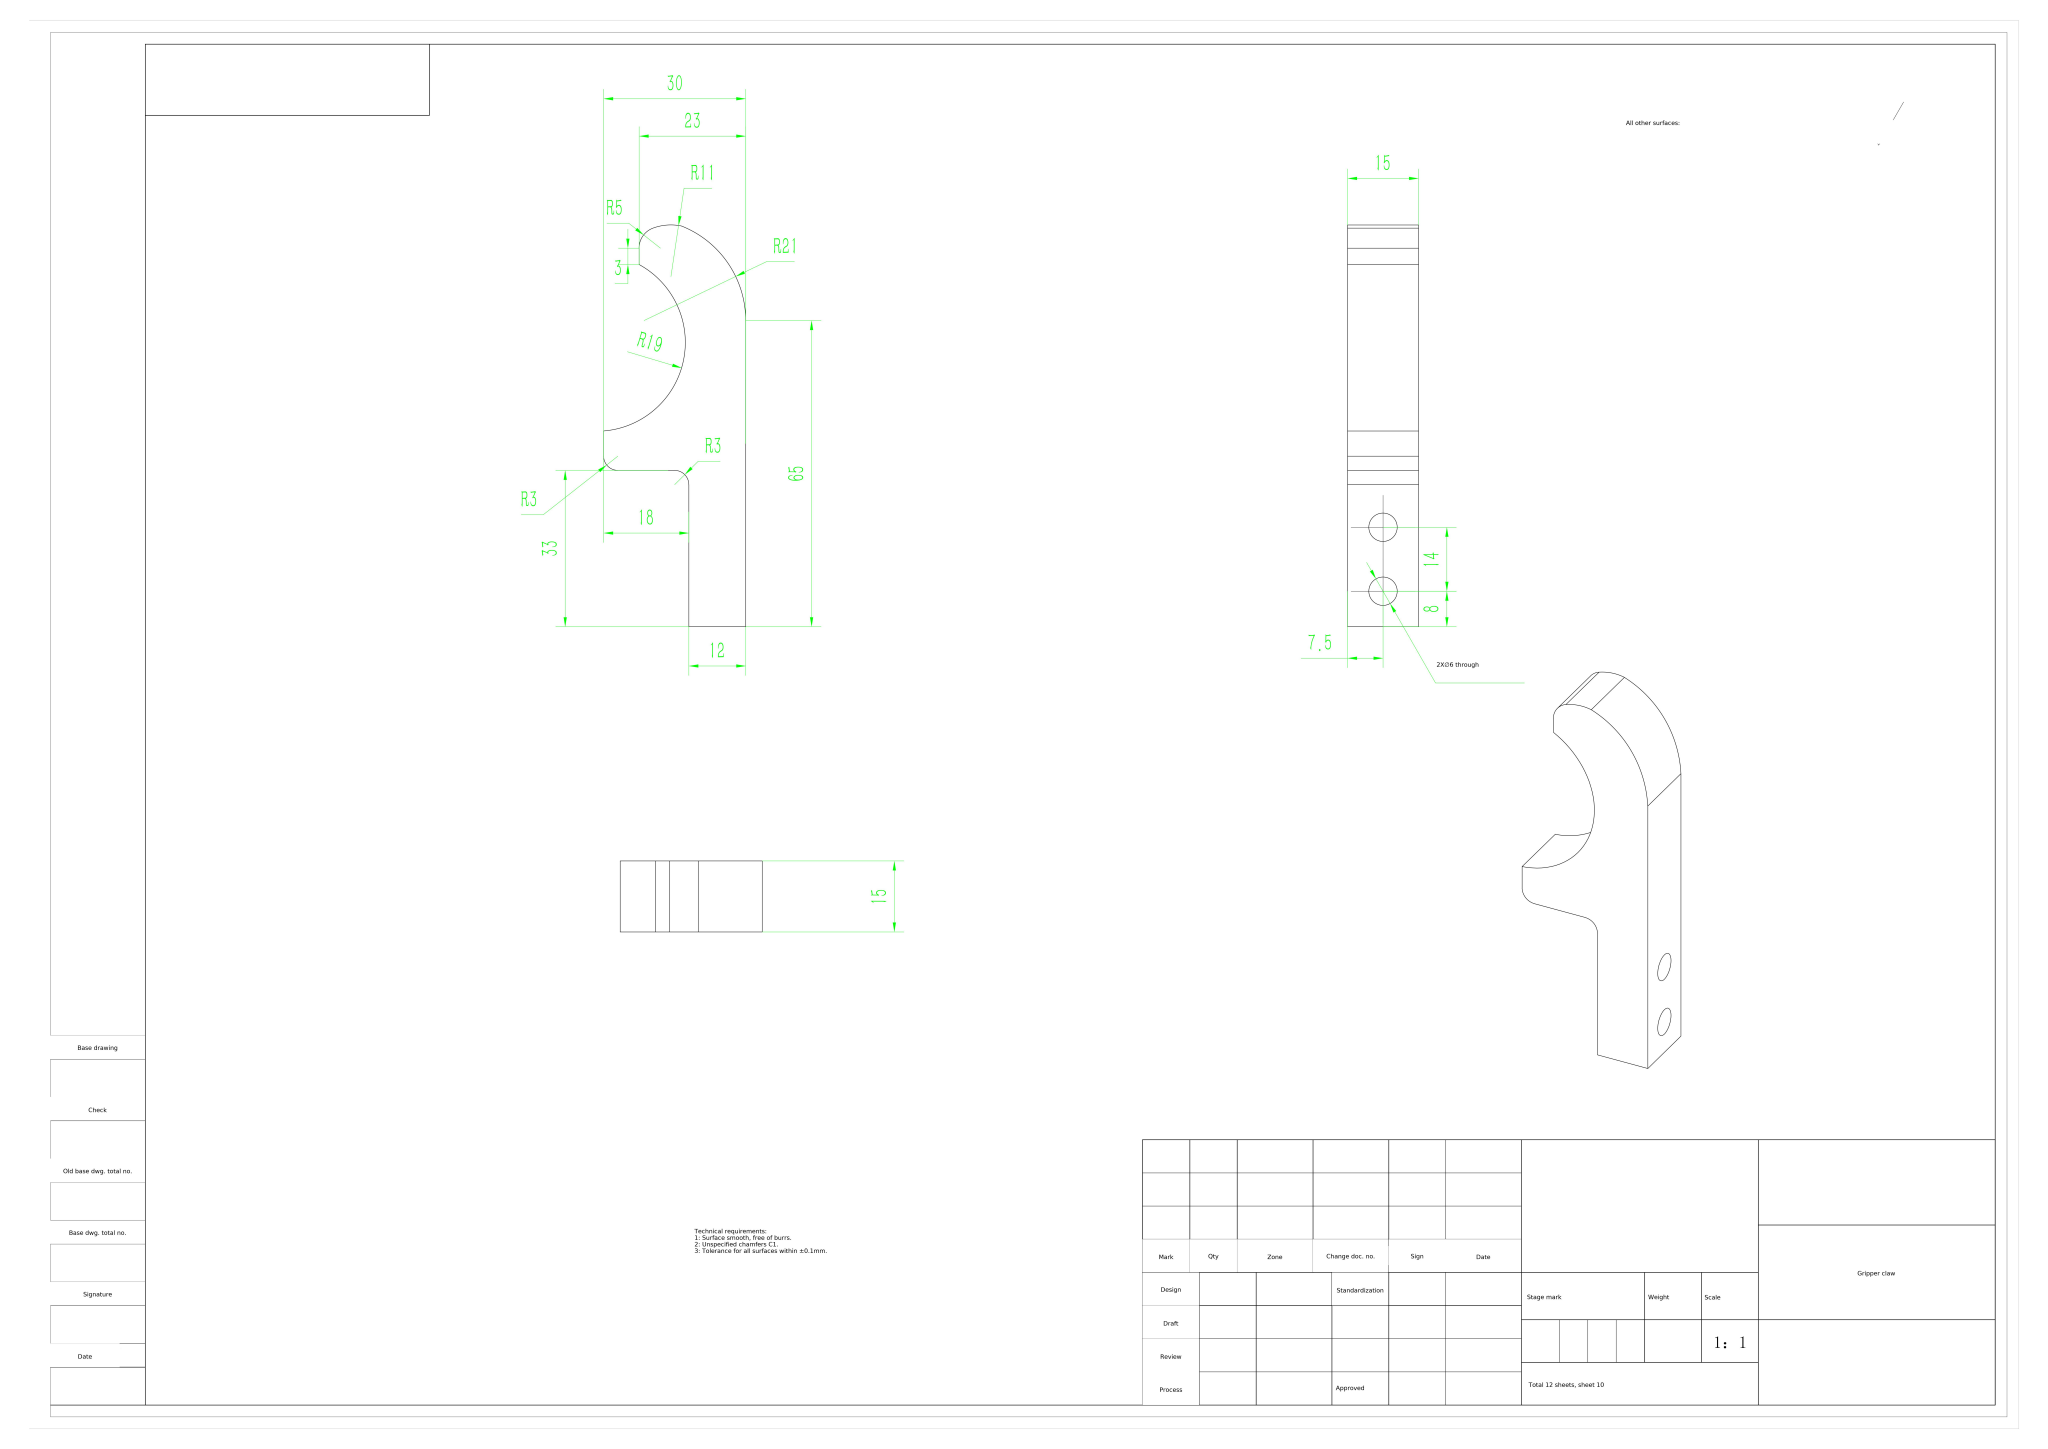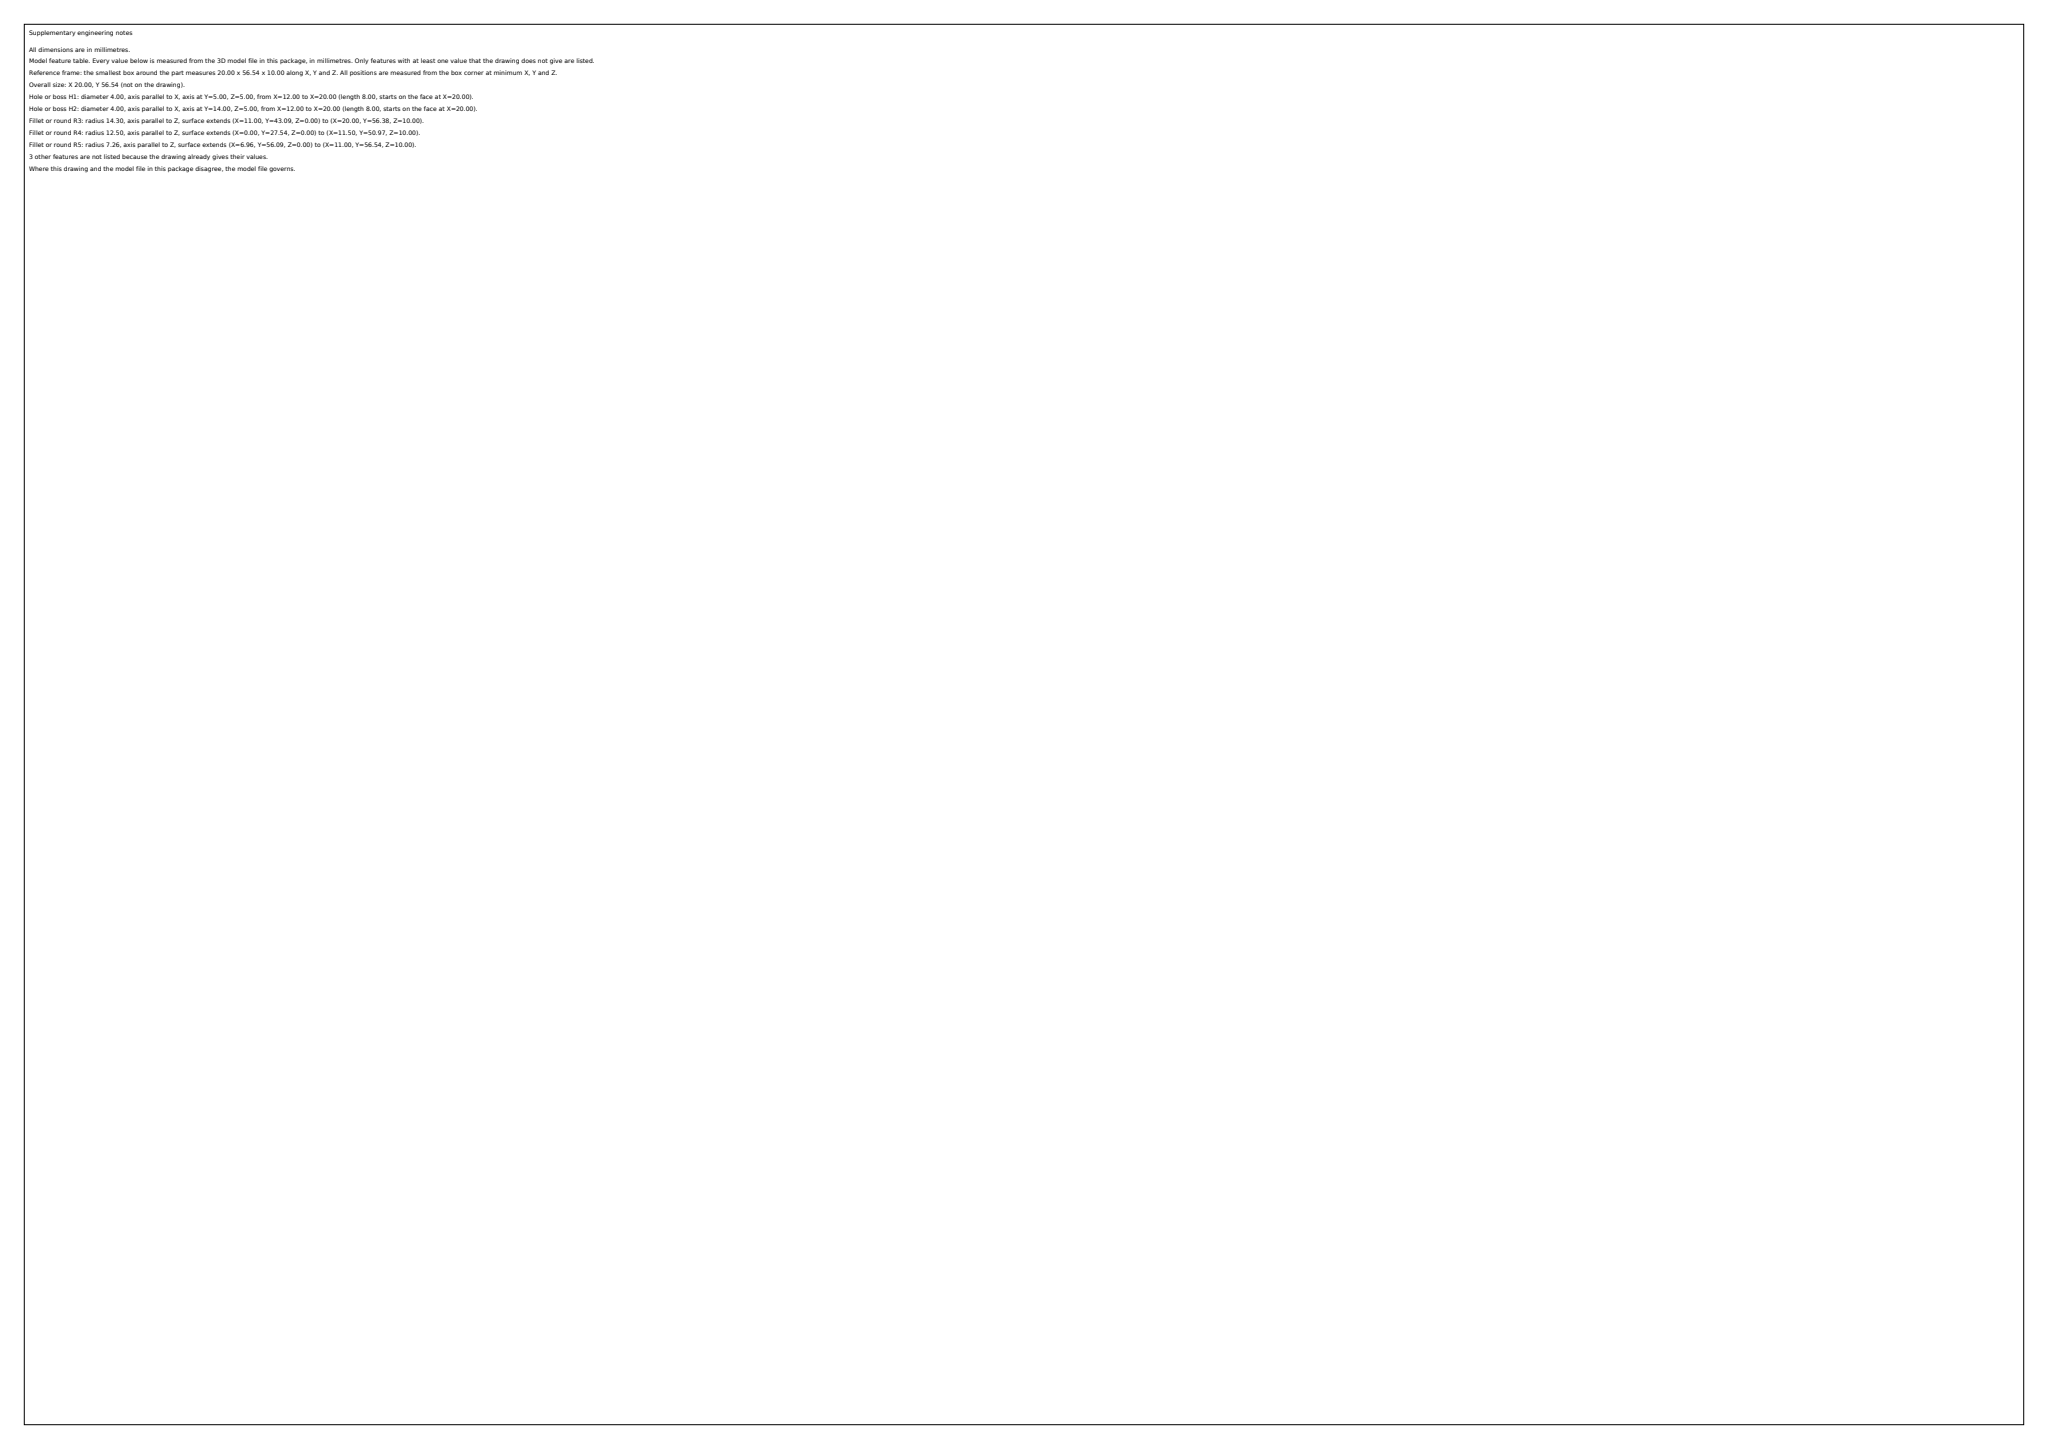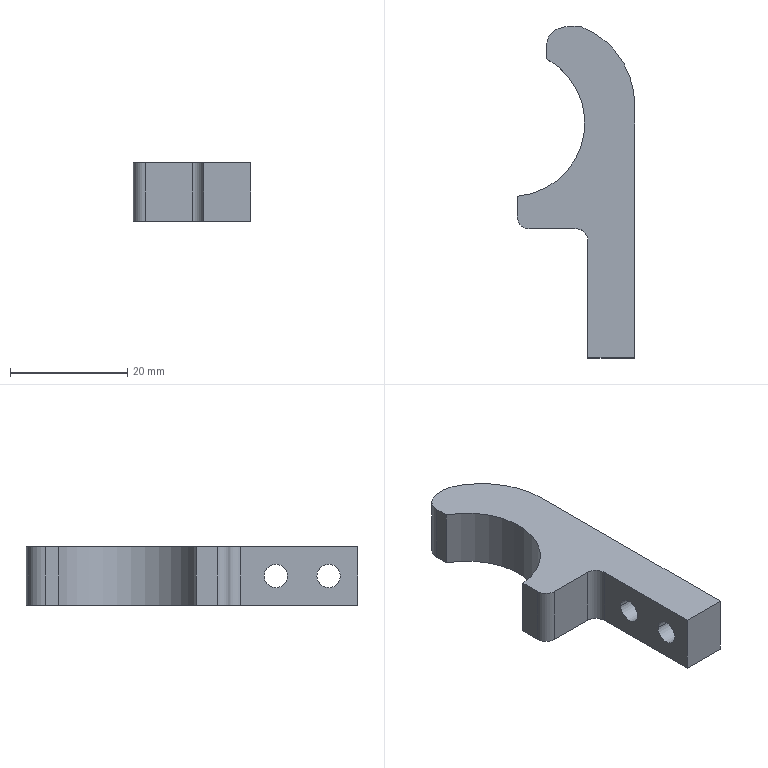Part | SolidWorks | mm | 1 solid | 18 faces | box 20 x 56.54 x 10 mm | volume 5658 mm3 | cylinder 10 | plane 8 | commonest cylinder face diameters 4 x6 14.515 x1 6 x1 25 x1 28.607 x1
STEP:
#1=CARTESIAN_POINT('',(21.,16.,0.));
#2=VERTEX_POINT('',#1);
#3=CARTESIAN_POINT('',(21.,12.,0.));
#4=VERTEX_POINT('',#3);
#5=CARTESIAN_POINT('',(21.,14.,0.));
#6=DIRECTION('',(-1.,-0.,0.));
#7=DIRECTION('',(0.,-1.,0.));
#8=AXIS2_PLACEMENT_3D('',#5,#6,#7);
#9=CIRCLE('',#8,2.);
#10=EDGE_CURVE('',#2,#4,#9,.T.);
#11=ORIENTED_EDGE('',*,*,#10,.F.);
#12=CARTESIAN_POINT('',(13.,16.,0.));
#13=VERTEX_POINT('',#12);
#14=CARTESIAN_POINT('',(21.,16.,0.));
#15=DIRECTION('',(-1.,-0.,0.));
#16=VECTOR('',#15,1000.);
#17=LINE('',#14,#16);
#18=EDGE_CURVE('',#2,#13,#17,.T.);
#19=ORIENTED_EDGE('',*,*,#18,.T.);
#20=CARTESIAN_POINT('',(13.,12.,0.));
#21=VERTEX_POINT('',#20);
#22=CARTESIAN_POINT('',(13.,14.,0.));
#23=DIRECTION('',(-1.,-0.,0.));
#24=DIRECTION('',(0.,-1.,0.));
#25=AXIS2_PLACEMENT_3D('',#22,#23,#24);
#26=CIRCLE('',#25,2.);
#27=EDGE_CURVE('',#13,#21,#26,.T.);
#28=ORIENTED_EDGE('',*,*,#27,.T.);
#29=CARTESIAN_POINT('',(21.,12.,0.));
#30=DIRECTION('',(-1.,-0.,0.));
#31=VECTOR('',#30,1000.);
#32=LINE('',#29,#31);
#33=EDGE_CURVE('',#4,#21,#32,.T.);
#34=ORIENTED_EDGE('',*,*,#33,.F.);
#35=EDGE_LOOP('',(#11,#19,#28,#34));
#36=FACE_OUTER_BOUND('',#35,.T.);
#37=CARTESIAN_POINT('',(21.,14.,0.));
#38=DIRECTION('',(-1.,-0.,0.));
#39=DIRECTION('',(0.,-1.,0.));
#40=AXIS2_PLACEMENT_3D('',#37,#38,#39);
#41=CYLINDRICAL_SURFACE('',#40,2.);
#42=ADVANCED_FACE('',(#36),#41,.F.);
#43=CARTESIAN_POINT('',(21.,7.,0.));
#44=VERTEX_POINT('',#43);
#45=CARTESIAN_POINT('',(21.,3.,0.));
#46=VERTEX_POINT('',#45);
#47=CARTESIAN_POINT('',(21.,5.,0.));
#48=DIRECTION('',(-1.,-0.,0.));
#49=DIRECTION('',(0.,-1.,0.));
#50=AXIS2_PLACEMENT_3D('',#47,#48,#49);
#51=CIRCLE('',#50,2.);
#52=EDGE_CURVE('',#44,#46,#51,.T.);
#53=ORIENTED_EDGE('',*,*,#52,.F.);
#54=CARTESIAN_POINT('',(13.,7.,0.));
#55=VERTEX_POINT('',#54);
#56=CARTESIAN_POINT('',(21.,7.,0.));
#57=DIRECTION('',(-1.,-0.,0.));
#58=VECTOR('',#57,1000.);
#59=LINE('',#56,#58);
#60=EDGE_CURVE('',#44,#55,#59,.T.);
#61=ORIENTED_EDGE('',*,*,#60,.T.);
#62=CARTESIAN_POINT('',(13.,3.,0.));
#63=VERTEX_POINT('',#62);
#64=CARTESIAN_POINT('',(13.,5.,0.));
#65=DIRECTION('',(-1.,-0.,0.));
#66=DIRECTION('',(0.,-1.,0.));
#67=AXIS2_PLACEMENT_3D('',#64,#65,#66);
#68=CIRCLE('',#67,2.);
#69=EDGE_CURVE('',#55,#63,#68,.T.);
#70=ORIENTED_EDGE('',*,*,#69,.T.);
#71=CARTESIAN_POINT('',(21.,3.,0.));
#72=DIRECTION('',(-1.,-0.,0.));
#73=VECTOR('',#72,1000.);
#74=LINE('',#71,#73);
#75=EDGE_CURVE('',#46,#63,#74,.T.);
#76=ORIENTED_EDGE('',*,*,#75,.F.);
#77=EDGE_LOOP('',(#53,#61,#70,#76));
#78=FACE_OUTER_BOUND('',#77,.T.);
#79=CARTESIAN_POINT('',(21.,5.,0.));
#80=DIRECTION('',(-1.,-0.,0.));
#81=DIRECTION('',(0.,-1.,0.));
#82=AXIS2_PLACEMENT_3D('',#79,#80,#81);
#83=CYLINDRICAL_SURFACE('',#82,2.);
#84=ADVANCED_FACE('',(#78),#83,.F.);
#85=CARTESIAN_POINT('',(7.965,56.094,-5.));
#86=VERTEX_POINT('',#85);
#87=CARTESIAN_POINT('',(12.,56.376,-5.));
#88=VERTEX_POINT('',#87);
#89=CARTESIAN_POINT('',(10.469,49.282,-5.));
#90=DIRECTION('',(0.,0.,-1.));
#91=DIRECTION('',(1.,0.,0.));
#92=AXIS2_PLACEMENT_3D('',#89,#90,#91);
#93=CIRCLE('',#92,7.257);
#94=EDGE_CURVE('',#86,#88,#93,.T.);
#95=ORIENTED_EDGE('',*,*,#94,.F.);
#96=CARTESIAN_POINT('',(7.965,56.094,5.));
#97=VERTEX_POINT('',#96);
#98=CARTESIAN_POINT('',(7.965,56.094,5.));
#99=DIRECTION('',(0.,0.,-1.));
#100=VECTOR('',#99,1000.);
#101=LINE('',#98,#100);
#102=EDGE_CURVE('',#97,#86,#101,.T.);
#103=ORIENTED_EDGE('',*,*,#102,.F.);
#104=CARTESIAN_POINT('',(12.,56.376,5.));
#105=VERTEX_POINT('',#104);
#106=CARTESIAN_POINT('',(10.469,49.282,5.));
#107=DIRECTION('',(0.,0.,-1.));
#108=DIRECTION('',(1.,0.,0.));
#109=AXIS2_PLACEMENT_3D('',#106,#107,#108);
#110=CIRCLE('',#109,7.257);
#111=EDGE_CURVE('',#97,#105,#110,.T.);
#112=ORIENTED_EDGE('',*,*,#111,.T.);
#113=CARTESIAN_POINT('',(12.,56.376,5.));
#114=DIRECTION('',(0.,0.,-1.));
#115=VECTOR('',#114,1000.);
#116=LINE('',#113,#115);
#117=EDGE_CURVE('',#105,#88,#116,.T.);
#118=ORIENTED_EDGE('',*,*,#117,.T.);
#119=EDGE_LOOP('',(#95,#103,#112,#118));
#120=FACE_OUTER_BOUND('',#119,.T.);
#121=CARTESIAN_POINT('',(10.469,49.282,5.));
#122=DIRECTION('',(0.,0.,-1.));
#123=DIRECTION('',(-1.,0.,0.));
#124=AXIS2_PLACEMENT_3D('',#121,#122,#123);
#125=CYLINDRICAL_SURFACE('',#124,7.257);
#126=ADVANCED_FACE('',(#120),#125,.T.);
#127=CARTESIAN_POINT('',(6.,53.278,-5.));
#128=VERTEX_POINT('',#127);
#129=CARTESIAN_POINT('',(9.,53.278,-5.));
#130=DIRECTION('',(0.,0.,1.));
#131=DIRECTION('',(1.,0.,0.));
#132=AXIS2_PLACEMENT_3D('',#129,#130,#131);
#133=CIRCLE('',#132,3.);
#134=EDGE_CURVE('',#86,#128,#133,.T.);
#135=ORIENTED_EDGE('',*,*,#134,.T.);
#136=CARTESIAN_POINT('',(6.,53.278,5.));
#137=VERTEX_POINT('',#136);
#138=CARTESIAN_POINT('',(6.,53.278,5.));
#139=DIRECTION('',(0.,0.,-1.));
#140=VECTOR('',#139,1000.);
#141=LINE('',#138,#140);
#142=EDGE_CURVE('',#137,#128,#141,.T.);
#143=ORIENTED_EDGE('',*,*,#142,.F.);
#144=CARTESIAN_POINT('',(9.,53.278,5.));
#145=DIRECTION('',(0.,0.,1.));
#146=DIRECTION('',(1.,0.,0.));
#147=AXIS2_PLACEMENT_3D('',#144,#145,#146);
#148=CIRCLE('',#147,3.);
#149=EDGE_CURVE('',#97,#137,#148,.T.);
#150=ORIENTED_EDGE('',*,*,#149,.F.);
#151=ORIENTED_EDGE('',*,*,#102,.T.);
#152=EDGE_LOOP('',(#135,#143,#150,#151));
#153=FACE_OUTER_BOUND('',#152,.T.);
#154=CARTESIAN_POINT('',(9.,53.278,5.));
#155=DIRECTION('',(0.,0.,-1.));
#156=DIRECTION('',(-1.,0.,0.));
#157=AXIS2_PLACEMENT_3D('',#154,#155,#156);
#158=CYLINDRICAL_SURFACE('',#157,3.);
#159=ADVANCED_FACE('',(#153),#158,.T.);
#160=CARTESIAN_POINT('',(6.,50.966,-5.));
#161=VERTEX_POINT('',#160);
#162=CARTESIAN_POINT('',(6.,0.,-5.));
#163=DIRECTION('',(0.,-1.,0.));
#164=VECTOR('',#163,1000.);
#165=LINE('',#162,#164);
#166=EDGE_CURVE('',#128,#161,#165,.T.);
#167=ORIENTED_EDGE('',*,*,#166,.T.);
#168=CARTESIAN_POINT('',(6.,50.966,5.));
#169=VERTEX_POINT('',#168);
#170=CARTESIAN_POINT('',(6.,50.966,5.));
#171=DIRECTION('',(0.,0.,-1.));
#172=VECTOR('',#171,1000.);
#173=LINE('',#170,#172);
#174=EDGE_CURVE('',#169,#161,#173,.T.);
#175=ORIENTED_EDGE('',*,*,#174,.F.);
#176=CARTESIAN_POINT('',(6.,0.,5.));
#177=DIRECTION('',(0.,-1.,0.));
#178=VECTOR('',#177,1000.);
#179=LINE('',#176,#178);
#180=EDGE_CURVE('',#137,#169,#179,.T.);
#181=ORIENTED_EDGE('',*,*,#180,.F.);
#182=ORIENTED_EDGE('',*,*,#142,.T.);
#183=EDGE_LOOP('',(#167,#175,#181,#182));
#184=FACE_OUTER_BOUND('',#183,.T.);
#185=CARTESIAN_POINT('',(6.,0.,5.));
#186=DIRECTION('',(1.,0.,0.));
#187=DIRECTION('',(0.,0.,-1.));
#188=AXIS2_PLACEMENT_3D('',#185,#186,#187);
#189=PLANE('',#188);
#190=ADVANCED_FACE('',(#184),#189,.F.);
#191=CARTESIAN_POINT('',(1.,27.54,-5.));
#192=VERTEX_POINT('',#191);
#193=CARTESIAN_POINT('',(0.,40.,-5.));
#194=DIRECTION('',(0.,0.,1.));
#195=DIRECTION('',(1.,0.,0.));
#196=AXIS2_PLACEMENT_3D('',#193,#194,#195);
#197=CIRCLE('',#196,12.5);
#198=EDGE_CURVE('',#192,#161,#197,.T.);
#199=ORIENTED_EDGE('',*,*,#198,.F.);
#200=CARTESIAN_POINT('',(1.,27.54,5.));
#201=VERTEX_POINT('',#200);
#202=CARTESIAN_POINT('',(1.,27.54,5.));
#203=DIRECTION('',(0.,0.,-1.));
#204=VECTOR('',#203,1000.);
#205=LINE('',#202,#204);
#206=EDGE_CURVE('',#201,#192,#205,.T.);
#207=ORIENTED_EDGE('',*,*,#206,.F.);
#208=CARTESIAN_POINT('',(0.,40.,5.));
#209=DIRECTION('',(0.,0.,1.));
#210=DIRECTION('',(1.,0.,0.));
#211=AXIS2_PLACEMENT_3D('',#208,#209,#210);
#212=CIRCLE('',#211,12.5);
#213=EDGE_CURVE('',#201,#169,#212,.T.);
#214=ORIENTED_EDGE('',*,*,#213,.T.);
#215=ORIENTED_EDGE('',*,*,#174,.T.);
#216=EDGE_LOOP('',(#199,#207,#214,#215));
#217=FACE_OUTER_BOUND('',#216,.T.);
#218=CARTESIAN_POINT('',(0.,40.,5.));
#219=DIRECTION('',(0.,0.,-1.));
#220=DIRECTION('',(-1.,0.,0.));
#221=AXIS2_PLACEMENT_3D('',#218,#219,#220);
#222=CYLINDRICAL_SURFACE('',#221,12.5);
#223=ADVANCED_FACE('',(#217),#222,.F.);
#224=CARTESIAN_POINT('',(1.,24.,-5.));
#225=VERTEX_POINT('',#224);
#226=CARTESIAN_POINT('',(1.,0.,-5.));
#227=DIRECTION('',(0.,-1.,0.));
#228=VECTOR('',#227,1000.);
#229=LINE('',#226,#228);
#230=EDGE_CURVE('',#192,#225,#229,.T.);
#231=ORIENTED_EDGE('',*,*,#230,.T.);
#232=CARTESIAN_POINT('',(1.,24.,5.));
#233=VERTEX_POINT('',#232);
#234=CARTESIAN_POINT('',(1.,24.,5.));
#235=DIRECTION('',(0.,0.,-1.));
#236=VECTOR('',#235,1000.);
#237=LINE('',#234,#236);
#238=EDGE_CURVE('',#233,#225,#237,.T.);
#239=ORIENTED_EDGE('',*,*,#238,.F.);
#240=CARTESIAN_POINT('',(1.,0.,5.));
#241=DIRECTION('',(0.,-1.,0.));
#242=VECTOR('',#241,1000.);
#243=LINE('',#240,#242);
#244=EDGE_CURVE('',#201,#233,#243,.T.);
#245=ORIENTED_EDGE('',*,*,#244,.F.);
#246=ORIENTED_EDGE('',*,*,#206,.T.);
#247=EDGE_LOOP('',(#231,#239,#245,#246));
#248=FACE_OUTER_BOUND('',#247,.T.);
#249=CARTESIAN_POINT('',(1.,0.,5.));
#250=DIRECTION('',(1.,0.,0.));
#251=DIRECTION('',(-0.,1.,0.));
#252=AXIS2_PLACEMENT_3D('',#249,#250,#251);
#253=PLANE('',#252);
#254=ADVANCED_FACE('',(#248),#253,.F.);
#255=CARTESIAN_POINT('',(3.,22.,-5.));
#256=VERTEX_POINT('',#255);
#257=CARTESIAN_POINT('',(3.,24.,-5.));
#258=DIRECTION('',(0.,0.,1.));
#259=DIRECTION('',(1.,0.,0.));
#260=AXIS2_PLACEMENT_3D('',#257,#258,#259);
#261=CIRCLE('',#260,2.);
#262=EDGE_CURVE('',#225,#256,#261,.T.);
#263=ORIENTED_EDGE('',*,*,#262,.T.);
#264=CARTESIAN_POINT('',(3.,22.,5.));
#265=VERTEX_POINT('',#264);
#266=CARTESIAN_POINT('',(3.,22.,5.));
#267=DIRECTION('',(0.,0.,-1.));
#268=VECTOR('',#267,1000.);
#269=LINE('',#266,#268);
#270=EDGE_CURVE('',#265,#256,#269,.T.);
#271=ORIENTED_EDGE('',*,*,#270,.F.);
#272=CARTESIAN_POINT('',(3.,24.,5.));
#273=DIRECTION('',(0.,0.,1.));
#274=DIRECTION('',(1.,0.,0.));
#275=AXIS2_PLACEMENT_3D('',#272,#273,#274);
#276=CIRCLE('',#275,2.);
#277=EDGE_CURVE('',#233,#265,#276,.T.);
#278=ORIENTED_EDGE('',*,*,#277,.F.);
#279=ORIENTED_EDGE('',*,*,#238,.T.);
#280=EDGE_LOOP('',(#263,#271,#278,#279));
#281=FACE_OUTER_BOUND('',#280,.T.);
#282=CARTESIAN_POINT('',(3.,24.,5.));
#283=DIRECTION('',(0.,0.,-1.));
#284=DIRECTION('',(-1.,0.,0.));
#285=AXIS2_PLACEMENT_3D('',#282,#283,#284);
#286=CYLINDRICAL_SURFACE('',#285,2.);
#287=ADVANCED_FACE('',(#281),#286,.T.);
#288=CARTESIAN_POINT('',(11.,22.,-5.));
#289=VERTEX_POINT('',#288);
#290=CARTESIAN_POINT('',(-0.,22.,-5.));
#291=DIRECTION('',(1.,0.,0.));
#292=VECTOR('',#291,1000.);
#293=LINE('',#290,#292);
#294=EDGE_CURVE('',#256,#289,#293,.T.);
#295=ORIENTED_EDGE('',*,*,#294,.T.);
#296=CARTESIAN_POINT('',(11.,22.,5.));
#297=VERTEX_POINT('',#296);
#298=CARTESIAN_POINT('',(11.,22.,5.));
#299=DIRECTION('',(0.,0.,-1.));
#300=VECTOR('',#299,1000.);
#301=LINE('',#298,#300);
#302=EDGE_CURVE('',#297,#289,#301,.T.);
#303=ORIENTED_EDGE('',*,*,#302,.F.);
#304=CARTESIAN_POINT('',(-0.,22.,5.));
#305=DIRECTION('',(1.,0.,0.));
#306=VECTOR('',#305,1000.);
#307=LINE('',#304,#306);
#308=EDGE_CURVE('',#265,#297,#307,.T.);
#309=ORIENTED_EDGE('',*,*,#308,.F.);
#310=ORIENTED_EDGE('',*,*,#270,.T.);
#311=EDGE_LOOP('',(#295,#303,#309,#310));
#312=FACE_OUTER_BOUND('',#311,.T.);
#313=CARTESIAN_POINT('',(-0.,22.,5.));
#314=DIRECTION('',(-0.,1.,0.));
#315=DIRECTION('',(-1.,-0.,0.));
#316=AXIS2_PLACEMENT_3D('',#313,#314,#315);
#317=PLANE('',#316);
#318=ADVANCED_FACE('',(#312),#317,.F.);
#319=CARTESIAN_POINT('',(13.,20.,-5.));
#320=VERTEX_POINT('',#319);
#321=CARTESIAN_POINT('',(11.,20.,-5.));
#322=DIRECTION('',(0.,0.,-1.));
#323=DIRECTION('',(1.,0.,0.));
#324=AXIS2_PLACEMENT_3D('',#321,#322,#323);
#325=CIRCLE('',#324,2.);
#326=EDGE_CURVE('',#289,#320,#325,.T.);
#327=ORIENTED_EDGE('',*,*,#326,.T.);
#328=CARTESIAN_POINT('',(13.,20.,5.));
#329=VERTEX_POINT('',#328);
#330=CARTESIAN_POINT('',(13.,20.,5.));
#331=DIRECTION('',(0.,0.,-1.));
#332=VECTOR('',#331,1000.);
#333=LINE('',#330,#332);
#334=EDGE_CURVE('',#329,#320,#333,.T.);
#335=ORIENTED_EDGE('',*,*,#334,.F.);
#336=CARTESIAN_POINT('',(11.,20.,5.));
#337=DIRECTION('',(0.,0.,-1.));
#338=DIRECTION('',(1.,0.,0.));
#339=AXIS2_PLACEMENT_3D('',#336,#337,#338);
#340=CIRCLE('',#339,2.);
#341=EDGE_CURVE('',#297,#329,#340,.T.);
#342=ORIENTED_EDGE('',*,*,#341,.F.);
#343=ORIENTED_EDGE('',*,*,#302,.T.);
#344=EDGE_LOOP('',(#327,#335,#342,#343));
#345=FACE_OUTER_BOUND('',#344,.T.);
#346=CARTESIAN_POINT('',(11.,20.,5.));
#347=DIRECTION('',(0.,0.,-1.));
#348=DIRECTION('',(-1.,0.,0.));
#349=AXIS2_PLACEMENT_3D('',#346,#347,#348);
#350=CYLINDRICAL_SURFACE('',#349,2.);
#351=ADVANCED_FACE('',(#345),#350,.F.);
#352=CARTESIAN_POINT('',(13.,14.,0.));
#353=DIRECTION('',(-1.,-0.,0.));
#354=DIRECTION('',(0.,-1.,0.));
#355=AXIS2_PLACEMENT_3D('',#352,#353,#354);
#356=CIRCLE('',#355,2.);
#357=EDGE_CURVE('',#21,#13,#356,.T.);
#358=ORIENTED_EDGE('',*,*,#357,.F.);
#359=ORIENTED_EDGE('',*,*,#27,.F.);
#360=EDGE_LOOP('',(#358,#359));
#361=FACE_BOUND('',#360,.T.);
#362=CARTESIAN_POINT('',(13.,5.,0.));
#363=DIRECTION('',(-1.,-0.,0.));
#364=DIRECTION('',(0.,-1.,0.));
#365=AXIS2_PLACEMENT_3D('',#362,#363,#364);
#366=CIRCLE('',#365,2.);
#367=EDGE_CURVE('',#63,#55,#366,.T.);
#368=ORIENTED_EDGE('',*,*,#367,.F.);
#369=ORIENTED_EDGE('',*,*,#69,.F.);
#370=EDGE_LOOP('',(#368,#369));
#371=FACE_BOUND('',#370,.T.);
#372=CARTESIAN_POINT('',(13.,-0.,-5.));
#373=VERTEX_POINT('',#372);
#374=CARTESIAN_POINT('',(13.,0.,-5.));
#375=DIRECTION('',(0.,-1.,0.));
#376=VECTOR('',#375,1000.);
#377=LINE('',#374,#376);
#378=EDGE_CURVE('',#320,#373,#377,.T.);
#379=ORIENTED_EDGE('',*,*,#378,.T.);
#380=CARTESIAN_POINT('',(13.,-0.,5.));
#381=VERTEX_POINT('',#380);
#382=CARTESIAN_POINT('',(13.,-0.,5.));
#383=DIRECTION('',(0.,0.,-1.));
#384=VECTOR('',#383,1000.);
#385=LINE('',#382,#384);
#386=EDGE_CURVE('',#381,#373,#385,.T.);
#387=ORIENTED_EDGE('',*,*,#386,.F.);
#388=CARTESIAN_POINT('',(13.,0.,5.));
#389=DIRECTION('',(0.,-1.,0.));
#390=VECTOR('',#389,1000.);
#391=LINE('',#388,#390);
#392=EDGE_CURVE('',#329,#381,#391,.T.);
#393=ORIENTED_EDGE('',*,*,#392,.F.);
#394=ORIENTED_EDGE('',*,*,#334,.T.);
#395=EDGE_LOOP('',(#379,#387,#393,#394));
#396=FACE_OUTER_BOUND('',#395,.T.);
#397=CARTESIAN_POINT('',(13.,0.,5.));
#398=DIRECTION('',(1.,0.,0.));
#399=DIRECTION('',(-0.,1.,0.));
#400=AXIS2_PLACEMENT_3D('',#397,#398,#399);
#401=PLANE('',#400);
#402=ADVANCED_FACE('',(#361,#371,#396),#401,.F.);
#403=CARTESIAN_POINT('',(21.,0.,-5.));
#404=VERTEX_POINT('',#403);
#405=CARTESIAN_POINT('',(0.,0.,-5.));
#406=DIRECTION('',(1.,0.,0.));
#407=VECTOR('',#406,1000.);
#408=LINE('',#405,#407);
#409=EDGE_CURVE('',#373,#404,#408,.T.);
#410=ORIENTED_EDGE('',*,*,#409,.T.);
#411=CARTESIAN_POINT('',(21.,0.,5.));
#412=VERTEX_POINT('',#411);
#413=CARTESIAN_POINT('',(21.,0.,5.));
#414=DIRECTION('',(0.,0.,-1.));
#415=VECTOR('',#414,1000.);
#416=LINE('',#413,#415);
#417=EDGE_CURVE('',#412,#404,#416,.T.);
#418=ORIENTED_EDGE('',*,*,#417,.F.);
#419=CARTESIAN_POINT('',(0.,0.,5.));
#420=DIRECTION('',(1.,0.,0.));
#421=VECTOR('',#420,1000.);
#422=LINE('',#419,#421);
#423=EDGE_CURVE('',#381,#412,#422,.T.);
#424=ORIENTED_EDGE('',*,*,#423,.F.);
#425=ORIENTED_EDGE('',*,*,#386,.T.);
#426=EDGE_LOOP('',(#410,#418,#424,#425));
#427=FACE_OUTER_BOUND('',#426,.T.);
#428=CARTESIAN_POINT('',(0.,0.,5.));
#429=DIRECTION('',(0.,1.,0.));
#430=DIRECTION('',(0.,0.,1.));
#431=AXIS2_PLACEMENT_3D('',#428,#429,#430);
#432=PLANE('',#431);
#433=ADVANCED_FACE('',(#427),#432,.F.);
#434=CARTESIAN_POINT('',(21.,14.,0.));
#435=DIRECTION('',(-1.,-0.,0.));
#436=DIRECTION('',(0.,-1.,0.));
#437=AXIS2_PLACEMENT_3D('',#434,#435,#436);
#438=CIRCLE('',#437,2.);
#439=EDGE_CURVE('',#4,#2,#438,.T.);
#440=ORIENTED_EDGE('',*,*,#439,.T.);
#441=ORIENTED_EDGE('',*,*,#10,.T.);
#442=EDGE_LOOP('',(#440,#441));
#443=FACE_BOUND('',#442,.T.);
#444=CARTESIAN_POINT('',(21.,5.,0.));
#445=DIRECTION('',(-1.,-0.,0.));
#446=DIRECTION('',(0.,-1.,0.));
#447=AXIS2_PLACEMENT_3D('',#444,#445,#446);
#448=CIRCLE('',#447,2.);
#449=EDGE_CURVE('',#46,#44,#448,.T.);
#450=ORIENTED_EDGE('',*,*,#449,.T.);
#451=ORIENTED_EDGE('',*,*,#52,.T.);
#452=EDGE_LOOP('',(#450,#451));
#453=FACE_BOUND('',#452,.T.);
#454=CARTESIAN_POINT('',(21.,43.092,-5.));
#455=VERTEX_POINT('',#454);
#456=CARTESIAN_POINT('',(21.,-0.,-5.));
#457=DIRECTION('',(0.,1.,0.));
#458=VECTOR('',#457,1000.);
#459=LINE('',#456,#458);
#460=EDGE_CURVE('',#404,#455,#459,.T.);
#461=ORIENTED_EDGE('',*,*,#460,.T.);
#462=CARTESIAN_POINT('',(21.,43.092,5.));
#463=VERTEX_POINT('',#462);
#464=CARTESIAN_POINT('',(21.,43.092,5.));
#465=DIRECTION('',(0.,0.,-1.));
#466=VECTOR('',#465,1000.);
#467=LINE('',#464,#466);
#468=EDGE_CURVE('',#463,#455,#467,.T.);
#469=ORIENTED_EDGE('',*,*,#468,.F.);
#470=CARTESIAN_POINT('',(21.,-0.,5.));
#471=DIRECTION('',(0.,1.,0.));
#472=VECTOR('',#471,1000.);
#473=LINE('',#470,#472);
#474=EDGE_CURVE('',#412,#463,#473,.T.);
#475=ORIENTED_EDGE('',*,*,#474,.F.);
#476=ORIENTED_EDGE('',*,*,#417,.T.);
#477=EDGE_LOOP('',(#461,#469,#475,#476));
#478=FACE_OUTER_BOUND('',#477,.T.);
#479=CARTESIAN_POINT('',(21.,-0.,5.));
#480=DIRECTION('',(-1.,0.,0.));
#481=DIRECTION('',(-0.,-1.,0.));
#482=AXIS2_PLACEMENT_3D('',#479,#480,#481);
#483=PLANE('',#482);
#484=ADVANCED_FACE('',(#443,#453,#478),#483,.F.);
#485=CARTESIAN_POINT('',(6.697,43.092,-5.));
#486=DIRECTION('',(0.,0.,-1.));
#487=DIRECTION('',(1.,-0.,0.));
#488=AXIS2_PLACEMENT_3D('',#485,#486,#487);
#489=CIRCLE('',#488,14.303);
#490=EDGE_CURVE('',#88,#455,#489,.T.);
#491=ORIENTED_EDGE('',*,*,#490,.F.);
#492=ORIENTED_EDGE('',*,*,#117,.F.);
#493=CARTESIAN_POINT('',(6.697,43.092,5.));
#494=DIRECTION('',(0.,0.,-1.));
#495=DIRECTION('',(1.,-0.,0.));
#496=AXIS2_PLACEMENT_3D('',#493,#494,#495);
#497=CIRCLE('',#496,14.303);
#498=EDGE_CURVE('',#105,#463,#497,.T.);
#499=ORIENTED_EDGE('',*,*,#498,.T.);
#500=ORIENTED_EDGE('',*,*,#468,.T.);
#501=EDGE_LOOP('',(#491,#492,#499,#500));
#502=FACE_OUTER_BOUND('',#501,.T.);
#503=CARTESIAN_POINT('',(6.697,43.092,5.));
#504=DIRECTION('',(0.,0.,-1.));
#505=DIRECTION('',(-1.,0.,0.));
#506=AXIS2_PLACEMENT_3D('',#503,#504,#505);
#507=CYLINDRICAL_SURFACE('',#506,14.303);
#508=ADVANCED_FACE('',(#502),#507,.T.);
#509=ORIENTED_EDGE('',*,*,#111,.F.);
#510=ORIENTED_EDGE('',*,*,#149,.T.);
#511=ORIENTED_EDGE('',*,*,#180,.T.);
#512=ORIENTED_EDGE('',*,*,#213,.F.);
#513=ORIENTED_EDGE('',*,*,#244,.T.);
#514=ORIENTED_EDGE('',*,*,#277,.T.);
#515=ORIENTED_EDGE('',*,*,#308,.T.);
#516=ORIENTED_EDGE('',*,*,#341,.T.);
#517=ORIENTED_EDGE('',*,*,#392,.T.);
#518=ORIENTED_EDGE('',*,*,#423,.T.);
#519=ORIENTED_EDGE('',*,*,#474,.T.);
#520=ORIENTED_EDGE('',*,*,#498,.F.);
#521=EDGE_LOOP('',(#509,#510,#511,#512,#513,#514,#515,#516,#517,#518,#519,#520));
#522=FACE_OUTER_BOUND('',#521,.T.);
#523=CARTESIAN_POINT('',(0.,0.,5.));
#524=DIRECTION('',(0.,0.,1.));
#525=DIRECTION('',(1.,0.,0.));
#526=AXIS2_PLACEMENT_3D('',#523,#524,#525);
#527=PLANE('',#526);
#528=ADVANCED_FACE('',(#522),#527,.T.);
#529=ORIENTED_EDGE('',*,*,#94,.T.);
#530=ORIENTED_EDGE('',*,*,#490,.T.);
#531=ORIENTED_EDGE('',*,*,#460,.F.);
#532=ORIENTED_EDGE('',*,*,#409,.F.);
#533=ORIENTED_EDGE('',*,*,#378,.F.);
#534=ORIENTED_EDGE('',*,*,#326,.F.);
#535=ORIENTED_EDGE('',*,*,#294,.F.);
#536=ORIENTED_EDGE('',*,*,#262,.F.);
#537=ORIENTED_EDGE('',*,*,#230,.F.);
#538=ORIENTED_EDGE('',*,*,#198,.T.);
#539=ORIENTED_EDGE('',*,*,#166,.F.);
#540=ORIENTED_EDGE('',*,*,#134,.F.);
#541=EDGE_LOOP('',(#529,#530,#531,#532,#533,#534,#535,#536,#537,#538,#539,#540));
#542=FACE_OUTER_BOUND('',#541,.T.);
#543=CARTESIAN_POINT('',(0.,0.,-5.));
#544=DIRECTION('',(0.,0.,1.));
#545=DIRECTION('',(1.,0.,0.));
#546=AXIS2_PLACEMENT_3D('',#543,#544,#545);
#547=PLANE('',#546);
#548=ADVANCED_FACE('',(#542),#547,.F.);
#549=ORIENTED_EDGE('',*,*,#60,.F.);
#550=ORIENTED_EDGE('',*,*,#449,.F.);
#551=ORIENTED_EDGE('',*,*,#75,.T.);
#552=ORIENTED_EDGE('',*,*,#367,.T.);
#553=EDGE_LOOP('',(#549,#550,#551,#552));
#554=FACE_OUTER_BOUND('',#553,.T.);
#555=CARTESIAN_POINT('',(21.,5.,0.));
#556=DIRECTION('',(-1.,-0.,0.));
#557=DIRECTION('',(0.,-1.,0.));
#558=AXIS2_PLACEMENT_3D('',#555,#556,#557);
#559=CYLINDRICAL_SURFACE('',#558,2.);
#560=ADVANCED_FACE('',(#554),#559,.F.);
#561=ORIENTED_EDGE('',*,*,#18,.F.);
#562=ORIENTED_EDGE('',*,*,#439,.F.);
#563=ORIENTED_EDGE('',*,*,#33,.T.);
#564=ORIENTED_EDGE('',*,*,#357,.T.);
#565=EDGE_LOOP('',(#561,#562,#563,#564));
#566=FACE_OUTER_BOUND('',#565,.T.);
#567=CARTESIAN_POINT('',(21.,14.,0.));
#568=DIRECTION('',(-1.,-0.,0.));
#569=DIRECTION('',(0.,-1.,0.));
#570=AXIS2_PLACEMENT_3D('',#567,#568,#569);
#571=CYLINDRICAL_SURFACE('',#570,2.);
#572=ADVANCED_FACE('',(#566),#571,.F.);
#573=CLOSED_SHELL('',(#42,#84,#126,#159,#190,#223,#254,#287,#318,#351,#402,#433,#484,#508,#528,#548,#560,#572));
#574=MANIFOLD_SOLID_BREP('',#573);
#575=CARTESIAN_POINT('',(0.,0.,0.));
#576=DIRECTION('',(0.,0.,1.));
#577=DIRECTION('',(1.,0.,0.));
#578=AXIS2_PLACEMENT_3D('',#575,#576,#577);
#579=(LENGTH_UNIT()NAMED_UNIT(*)SI_UNIT(.MILLI.,.METRE.));
#580=UNCERTAINTY_MEASURE_WITH_UNIT(LENGTH_MEASURE(0.00001),#579,'','');
#581=(NAMED_UNIT(*)PLANE_ANGLE_UNIT()SI_UNIT($,.RADIAN.));
#582=(NAMED_UNIT(*)SI_UNIT($,.STERADIAN.)SOLID_ANGLE_UNIT());
#583=(GEOMETRIC_REPRESENTATION_CONTEXT(3)GLOBAL_UNCERTAINTY_ASSIGNED_CONTEXT((#580))GLOBAL_UNIT_ASSIGNED_CONTEXT((#579,#581,#582))REPRESENTATION_CONTEXT('',''));
#584=ADVANCED_BREP_SHAPE_REPRESENTATION('',(#574,#578),#583);